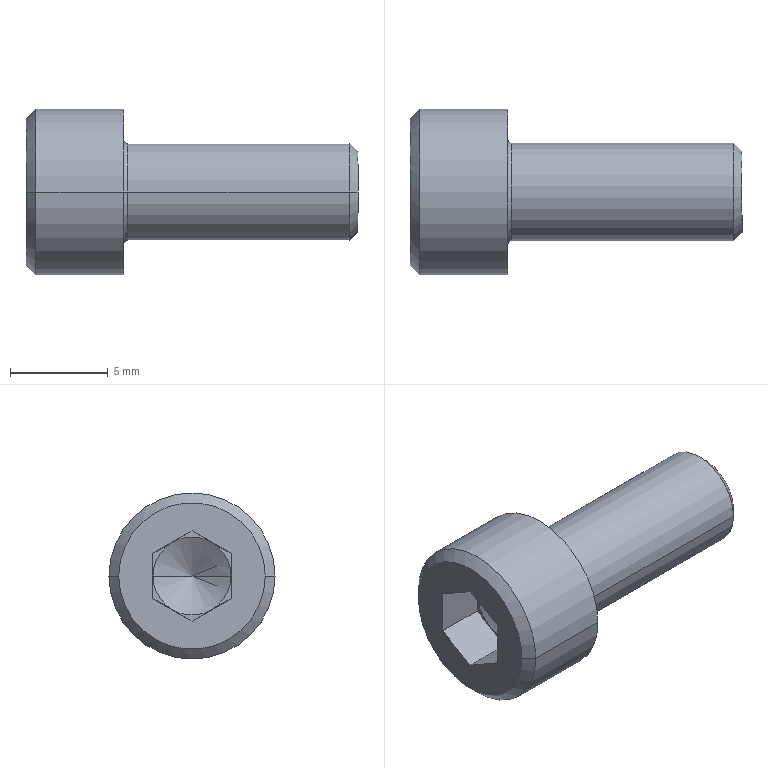Component | SolidWorks | ServoDriveMotorModule-1_MCOCGWK38_16_16-1_M5-1 | 1 solid | 27 faces | box 17 x 8.5 x 8.5 mm | volume 475 mm3 | plane 15 | cone 6 | cylinder 4 | torus 2 | commonest cylinder face diameters 8.5 x2 5 x2 | material AISI 1045 Steel, cold drawn
build123d program:
from build123d import *

# Parameters (mm, degrees)
CUT_EXTRUDE1_DEPTH = 2.5


with BuildPart() as part:
    # Sketch1 → Revolve1 (revolve)
    with BuildSketch(Plane.XY, mode=Mode.PRIVATE) as revolve1_sk:
        with BuildLine():
            Line((-5, 0), (-5, 3.75))
            Line((-5, 3.75), (-4.5, 4.25))
            Line((-4.5, 4.25), (0, 4.25))
            Line((0, 4.25), (0, 2.7))
            ThreePointArc((0, 2.7), (0.05858, 2.559), (0.2, 2.5))
            Line((0.2, 2.5), (11.567, 2.5))
            Line((11.567, 2.5), (12, 2.067))
            Line((12, 2.067), (12, 0))
            Line((12, 0), (-5, 0))
        make_face()
    revolve(revolve1_sk.sketch.rotate(Axis((12, 0, 0), (-1, 0, 0)), 270), axis=Axis((12, 0, 0), (-1, 0, 0)))

    # Sketch2 → Cut-Extrude1 (cut)
    with BuildSketch(Plane(origin=(-5, 0, 0), x_dir=(0, 0, -1), z_dir=(1, 0, 0))):
        Polygon((-2, 1.155), (-2, -1.155), (0, -2.309), (2, -1.155), (2, 1.155), (0, 2.309), align=None)
    extrude(amount=CUT_EXTRUDE1_DEPTH, mode=Mode.SUBTRACT)

    # Sketch3 → Cut-Revolve1 (revolve, cut)
    with BuildSketch(Plane.XY, mode=Mode.PRIVATE) as cut_revolve1_sk:
        Polygon((-2.5, 0), (-2.5, 2), (-1.345, 0), align=None)
    revolve(cut_revolve1_sk.sketch.rotate(Axis((-1.345, 0, 0), (-1, 0, 0)), 270), axis=Axis((-1.345, 0, 0), (-1, 0, 0)), mode=Mode.SUBTRACT)


solid = part.part

# Placed as in the assembly
solid = solid.moved(Location((-8.4, -11.5, 109), (90, 0, 0)))
STEP:
#1=COLOUR_RGB('',0.7922,0.8196,0.9333);
#2=FILL_AREA_STYLE_COLOUR('',#1);
#3=FILL_AREA_STYLE('',(#2));
#4=SURFACE_STYLE_FILL_AREA(#3);
#5=SURFACE_SIDE_STYLE('',(#4));
#6=SURFACE_STYLE_USAGE(.BOTH.,#5);
#7=PRESENTATION_STYLE_ASSIGNMENT((#6));
#8=CARTESIAN_POINT('',(-0.3837,-0.4528,4.291));
#9=VERTEX_POINT('',#8);
#10=CARTESIAN_POINT('',(-0.4291,-0.374,4.291));
#11=VERTEX_POINT('',#10);
#12=CARTESIAN_POINT('',(-0.3837,-0.4528,4.291));
#13=DIRECTION('',(-0.5,0.866,0.));
#14=VECTOR('',#13,39.37);
#15=LINE('',#12,#14);
#16=EDGE_CURVE('',#9,#11,#15,.T.);
#17=ORIENTED_EDGE('',*,*,#16,.F.);
#18=CARTESIAN_POINT('',(-0.4291,-0.5315,4.291));
#19=VERTEX_POINT('',#18);
#20=CARTESIAN_POINT('',(-0.3837,-0.4528,4.291));
#21=DIRECTION('',(-0.5,-0.866,-0.));
#22=VECTOR('',#21,39.37);
#23=LINE('',#20,#22);
#24=EDGE_CURVE('',#9,#19,#23,.T.);
#25=ORIENTED_EDGE('',*,*,#24,.T.);
#26=CARTESIAN_POINT('',(-0.4291,-0.4921,4.36));
#27=VERTEX_POINT('',#26);
#28=CARTESIAN_POINT('',(-0.4291,-0.4528,4.291));
#29=DIRECTION('',(-1.,-0.,0.));
#30=DIRECTION('',(-0.,1.,0.));
#31=AXIS2_PLACEMENT_3D('',#28,#29,#30);
#32=CIRCLE('',#31,0.07874);
#33=EDGE_CURVE('',#19,#27,#32,.T.);
#34=ORIENTED_EDGE('',*,*,#33,.T.);
#35=CARTESIAN_POINT('',(-0.4291,-0.4134,4.36));
#36=VERTEX_POINT('',#35);
#37=CARTESIAN_POINT('',(-0.4291,-0.4528,4.291));
#38=DIRECTION('',(-1.,-0.,0.));
#39=DIRECTION('',(-0.,1.,0.));
#40=AXIS2_PLACEMENT_3D('',#37,#38,#39);
#41=CIRCLE('',#40,0.07874);
#42=EDGE_CURVE('',#27,#36,#41,.T.);
#43=ORIENTED_EDGE('',*,*,#42,.T.);
#44=CARTESIAN_POINT('',(-0.4291,-0.4528,4.291));
#45=DIRECTION('',(-1.,-0.,0.));
#46=DIRECTION('',(-0.,1.,0.));
#47=AXIS2_PLACEMENT_3D('',#44,#45,#46);
#48=CIRCLE('',#47,0.07874);
#49=EDGE_CURVE('',#36,#11,#48,.T.);
#50=ORIENTED_EDGE('',*,*,#49,.T.);
#51=EDGE_LOOP('',(#17,#25,#34,#43,#50));
#52=FACE_OUTER_BOUND('',#51,.T.);
#53=CARTESIAN_POINT('',(-39.754,-0.4528,4.291));
#54=DIRECTION('',(-1.,-0.,0.));
#55=DIRECTION('',(-0.,1.,0.));
#56=AXIS2_PLACEMENT_3D('',#53,#54,#55);
#57=CONICAL_SURFACE('',#56,68.191,1.047);
#58=ADVANCED_FACE('',(#52),#57,.F.);
#59=CARTESIAN_POINT('',(-0.5276,-0.3051,4.291));
#60=VERTEX_POINT('',#59);
#61=CARTESIAN_POINT('',(-0.5276,-0.6004,4.291));
#62=VERTEX_POINT('',#61);
#63=CARTESIAN_POINT('',(-0.5276,-0.4528,4.291));
#64=DIRECTION('',(-1.,-0.,0.));
#65=DIRECTION('',(-0.,1.,0.));
#66=AXIS2_PLACEMENT_3D('',#63,#64,#65);
#67=CIRCLE('',#66,0.1476);
#68=EDGE_CURVE('',#60,#62,#67,.T.);
#69=ORIENTED_EDGE('',*,*,#68,.F.);
#70=CARTESIAN_POINT('',(-0.5079,-0.2854,4.291));
#71=VERTEX_POINT('',#70);
#72=CARTESIAN_POINT('',(-0.5079,-0.2854,4.291));
#73=DIRECTION('',(0.7071,0.7071,-0.));
#74=VECTOR('',#73,39.37);
#75=LINE('',#72,#74);
#76=EDGE_CURVE('',#60,#71,#75,.T.);
#77=ORIENTED_EDGE('',*,*,#76,.T.);
#78=CARTESIAN_POINT('',(-0.5079,-0.6201,4.291));
#79=VERTEX_POINT('',#78);
#80=CARTESIAN_POINT('',(-0.5079,-0.4528,4.291));
#81=DIRECTION('',(-1.,-0.,0.));
#82=DIRECTION('',(-0.,1.,0.));
#83=AXIS2_PLACEMENT_3D('',#80,#81,#82);
#84=CIRCLE('',#83,0.1673);
#85=EDGE_CURVE('',#71,#79,#84,.T.);
#86=ORIENTED_EDGE('',*,*,#85,.T.);
#87=CARTESIAN_POINT('',(-0.5079,-0.6201,4.291));
#88=DIRECTION('',(0.7071,-0.7071,-0.));
#89=VECTOR('',#88,39.37);
#90=LINE('',#87,#89);
#91=EDGE_CURVE('',#62,#79,#90,.T.);
#92=ORIENTED_EDGE('',*,*,#91,.F.);
#93=EDGE_LOOP('',(#69,#77,#86,#92));
#94=FACE_OUTER_BOUND('',#93,.T.);
#95=CARTESIAN_POINT('',(-0.5079,-0.4528,4.291));
#96=DIRECTION('',(1.,0.,-0.));
#97=DIRECTION('',(0.,-1.,0.));
#98=AXIS2_PLACEMENT_3D('',#95,#96,#97);
#99=CONICAL_SURFACE('',#98,0.1673,0.7854);
#100=ADVANCED_FACE('',(#94),#99,.T.);
#101=CARTESIAN_POINT('',(-0.3307,-0.2854,4.291));
#102=VERTEX_POINT('',#101);
#103=CARTESIAN_POINT('',(-0.3307,-0.6201,4.291));
#104=VERTEX_POINT('',#103);
#105=CARTESIAN_POINT('',(-0.3307,-0.4528,4.291));
#106=DIRECTION('',(-1.,-0.,0.));
#107=DIRECTION('',(-0.,1.,0.));
#108=AXIS2_PLACEMENT_3D('',#105,#106,#107);
#109=CIRCLE('',#108,0.1673);
#110=EDGE_CURVE('',#102,#104,#109,.T.);
#111=ORIENTED_EDGE('',*,*,#110,.T.);
#112=CARTESIAN_POINT('',(0.1417,-0.6201,4.291));
#113=DIRECTION('',(-1.,-0.,0.));
#114=VECTOR('',#113,39.37);
#115=LINE('',#112,#114);
#116=EDGE_CURVE('',#104,#79,#115,.T.);
#117=ORIENTED_EDGE('',*,*,#116,.T.);
#118=ORIENTED_EDGE('',*,*,#85,.F.);
#119=CARTESIAN_POINT('',(0.1417,-0.2854,4.291));
#120=DIRECTION('',(-1.,-0.,0.));
#121=VECTOR('',#120,39.37);
#122=LINE('',#119,#121);
#123=EDGE_CURVE('',#102,#71,#122,.T.);
#124=ORIENTED_EDGE('',*,*,#123,.F.);
#125=EDGE_LOOP('',(#111,#117,#118,#124));
#126=FACE_OUTER_BOUND('',#125,.T.);
#127=CARTESIAN_POINT('',(0.1417,-0.4528,4.291));
#128=DIRECTION('',(-1.,-0.,0.));
#129=DIRECTION('',(-0.,1.,0.));
#130=AXIS2_PLACEMENT_3D('',#127,#128,#129);
#131=CYLINDRICAL_SURFACE('',#130,0.1673);
#132=ADVANCED_FACE('',(#126),#131,.T.);
#133=CARTESIAN_POINT('',(-0.3307,-0.5591,4.291));
#134=VERTEX_POINT('',#133);
#135=CARTESIAN_POINT('',(-0.3307,-0.3465,4.291));
#136=VERTEX_POINT('',#135);
#137=CARTESIAN_POINT('',(-0.3307,-0.4528,4.291));
#138=DIRECTION('',(-1.,-0.,0.));
#139=DIRECTION('',(-0.,1.,0.));
#140=AXIS2_PLACEMENT_3D('',#137,#138,#139);
#141=CIRCLE('',#140,0.1063);
#142=EDGE_CURVE('',#134,#136,#141,.T.);
#143=ORIENTED_EDGE('',*,*,#142,.F.);
#144=CARTESIAN_POINT('',(-0.3228,-0.5512,4.291));
#145=VERTEX_POINT('',#144);
#146=CARTESIAN_POINT('',(-0.3228,-0.5591,4.291));
#147=DIRECTION('',(-0.,0.,-1.));
#148=DIRECTION('',(0.,1.,0.));
#149=AXIS2_PLACEMENT_3D('',#146,#147,#148);
#150=CIRCLE('',#149,0.007874);
#151=EDGE_CURVE('',#134,#145,#150,.T.);
#152=ORIENTED_EDGE('',*,*,#151,.T.);
#153=CARTESIAN_POINT('',(-0.3228,-0.3543,4.291));
#154=VERTEX_POINT('',#153);
#155=CARTESIAN_POINT('',(-0.3228,-0.4528,4.291));
#156=DIRECTION('',(-1.,-0.,0.));
#157=DIRECTION('',(-0.,1.,0.));
#158=AXIS2_PLACEMENT_3D('',#155,#156,#157);
#159=CIRCLE('',#158,0.09843);
#160=EDGE_CURVE('',#145,#154,#159,.T.);
#161=ORIENTED_EDGE('',*,*,#160,.T.);
#162=CARTESIAN_POINT('',(-0.3228,-0.3465,4.291));
#163=DIRECTION('',(0.,-0.,1.));
#164=DIRECTION('',(1.,0.,0.));
#165=AXIS2_PLACEMENT_3D('',#162,#163,#164);
#166=CIRCLE('',#165,0.007874);
#167=EDGE_CURVE('',#136,#154,#166,.T.);
#168=ORIENTED_EDGE('',*,*,#167,.F.);
#169=EDGE_LOOP('',(#143,#152,#161,#168));
#170=FACE_OUTER_BOUND('',#169,.T.);
#171=CARTESIAN_POINT('',(-0.3228,-0.4528,4.291));
#172=DIRECTION('',(-1.,-0.,0.));
#173=DIRECTION('',(-0.,1.,-0.));
#174=AXIS2_PLACEMENT_3D('',#171,#172,#173);
#175=TOROIDAL_SURFACE('',#174,0.1063,0.007874);
#176=ADVANCED_FACE('',(#170),#175,.F.);
#177=CARTESIAN_POINT('',(0.1247,-0.3543,4.291));
#178=VERTEX_POINT('',#177);
#179=CARTESIAN_POINT('',(0.1247,-0.5512,4.291));
#180=VERTEX_POINT('',#179);
#181=CARTESIAN_POINT('',(0.1247,-0.4528,4.291));
#182=DIRECTION('',(-1.,-0.,0.));
#183=DIRECTION('',(-0.,1.,0.));
#184=AXIS2_PLACEMENT_3D('',#181,#182,#183);
#185=CIRCLE('',#184,0.09843);
#186=EDGE_CURVE('',#178,#180,#185,.T.);
#187=ORIENTED_EDGE('',*,*,#186,.T.);
#188=CARTESIAN_POINT('',(0.1417,-0.5512,4.291));
#189=DIRECTION('',(-1.,-0.,0.));
#190=VECTOR('',#189,39.37);
#191=LINE('',#188,#190);
#192=EDGE_CURVE('',#180,#145,#191,.T.);
#193=ORIENTED_EDGE('',*,*,#192,.T.);
#194=CARTESIAN_POINT('',(-0.3228,-0.4528,4.291));
#195=DIRECTION('',(-1.,-0.,0.));
#196=DIRECTION('',(-0.,1.,0.));
#197=AXIS2_PLACEMENT_3D('',#194,#195,#196);
#198=CIRCLE('',#197,0.09843);
#199=EDGE_CURVE('',#154,#145,#198,.T.);
#200=ORIENTED_EDGE('',*,*,#199,.F.);
#201=CARTESIAN_POINT('',(0.1417,-0.3543,4.291));
#202=DIRECTION('',(-1.,-0.,0.));
#203=VECTOR('',#202,39.37);
#204=LINE('',#201,#203);
#205=EDGE_CURVE('',#178,#154,#204,.T.);
#206=ORIENTED_EDGE('',*,*,#205,.F.);
#207=EDGE_LOOP('',(#187,#193,#200,#206));
#208=FACE_OUTER_BOUND('',#207,.T.);
#209=CARTESIAN_POINT('',(0.1417,-0.4528,4.291));
#210=DIRECTION('',(-1.,-0.,0.));
#211=DIRECTION('',(-0.,1.,0.));
#212=AXIS2_PLACEMENT_3D('',#209,#210,#211);
#213=CYLINDRICAL_SURFACE('',#212,0.09843);
#214=ADVANCED_FACE('',(#208),#213,.T.);
#215=CARTESIAN_POINT('',(0.1417,-0.3714,4.291));
#216=VERTEX_POINT('',#215);
#217=CARTESIAN_POINT('',(0.1417,-0.5341,4.291));
#218=VERTEX_POINT('',#217);
#219=CARTESIAN_POINT('',(0.1417,-0.4528,4.291));
#220=DIRECTION('',(-1.,-0.,0.));
#221=DIRECTION('',(-0.,1.,0.));
#222=AXIS2_PLACEMENT_3D('',#219,#220,#221);
#223=CIRCLE('',#222,0.08138);
#224=EDGE_CURVE('',#216,#218,#223,.T.);
#225=ORIENTED_EDGE('',*,*,#224,.T.);
#226=CARTESIAN_POINT('',(0.1417,-0.5341,4.291));
#227=DIRECTION('',(-0.7071,-0.7071,-0.));
#228=VECTOR('',#227,39.37);
#229=LINE('',#226,#228);
#230=EDGE_CURVE('',#218,#180,#229,.T.);
#231=ORIENTED_EDGE('',*,*,#230,.T.);
#232=ORIENTED_EDGE('',*,*,#186,.F.);
#233=CARTESIAN_POINT('',(0.1417,-0.3714,4.291));
#234=DIRECTION('',(-0.7071,0.7071,0.));
#235=VECTOR('',#234,39.37);
#236=LINE('',#233,#235);
#237=EDGE_CURVE('',#216,#178,#236,.T.);
#238=ORIENTED_EDGE('',*,*,#237,.F.);
#239=EDGE_LOOP('',(#225,#231,#232,#238));
#240=FACE_OUTER_BOUND('',#239,.T.);
#241=CARTESIAN_POINT('',(0.1417,-0.4528,4.291));
#242=DIRECTION('',(-1.,-0.,0.));
#243=DIRECTION('',(-0.,1.,0.));
#244=AXIS2_PLACEMENT_3D('',#241,#242,#243);
#245=CONICAL_SURFACE('',#244,0.08138,0.7854);
#246=ADVANCED_FACE('',(#240),#245,.T.);
#247=CARTESIAN_POINT('',(-0.4291,-0.4134,4.223));
#248=VERTEX_POINT('',#247);
#249=CARTESIAN_POINT('',(-0.4291,-0.4528,4.291));
#250=DIRECTION('',(-1.,-0.,0.));
#251=DIRECTION('',(-0.,1.,0.));
#252=AXIS2_PLACEMENT_3D('',#249,#250,#251);
#253=CIRCLE('',#252,0.07874);
#254=EDGE_CURVE('',#11,#248,#253,.T.);
#255=ORIENTED_EDGE('',*,*,#254,.F.);
#256=CARTESIAN_POINT('',(-0.4291,-0.374,4.246));
#257=VERTEX_POINT('',#256);
#258=CARTESIAN_POINT('',(-0.4291,-0.374,4.246));
#259=DIRECTION('',(0.,-0.,1.));
#260=VECTOR('',#259,39.37);
#261=LINE('',#258,#260);
#262=EDGE_CURVE('',#257,#11,#261,.T.);
#263=ORIENTED_EDGE('',*,*,#262,.F.);
#264=CARTESIAN_POINT('',(-0.4291,-0.4528,4.2));
#265=DIRECTION('',(-0.,0.866,0.5));
#266=VECTOR('',#265,39.37);
#267=LINE('',#264,#266);
#268=EDGE_CURVE('',#248,#257,#267,.T.);
#269=ORIENTED_EDGE('',*,*,#268,.F.);
#270=EDGE_LOOP('',(#255,#263,#269));
#271=FACE_OUTER_BOUND('',#270,.T.);
#272=CARTESIAN_POINT('',(-0.4291,-0.4528,4.291));
#273=DIRECTION('',(1.,0.,-0.));
#274=DIRECTION('',(0.,-1.,-0.));
#275=AXIS2_PLACEMENT_3D('',#272,#273,#274);
#276=PLANE('',#275);
#277=ADVANCED_FACE('',(#271),#276,.F.);
#278=CARTESIAN_POINT('',(-0.4291,-0.4921,4.223));
#279=VERTEX_POINT('',#278);
#280=CARTESIAN_POINT('',(-0.4291,-0.4528,4.291));
#281=DIRECTION('',(-1.,-0.,0.));
#282=DIRECTION('',(-0.,1.,0.));
#283=AXIS2_PLACEMENT_3D('',#280,#281,#282);
#284=CIRCLE('',#283,0.07874);
#285=EDGE_CURVE('',#248,#279,#284,.T.);
#286=ORIENTED_EDGE('',*,*,#285,.F.);
#287=CARTESIAN_POINT('',(-0.4291,-0.4528,4.2));
#288=VERTEX_POINT('',#287);
#289=CARTESIAN_POINT('',(-0.4291,-0.4528,4.2));
#290=DIRECTION('',(-0.,0.866,0.5));
#291=VECTOR('',#290,39.37);
#292=LINE('',#289,#291);
#293=EDGE_CURVE('',#288,#248,#292,.T.);
#294=ORIENTED_EDGE('',*,*,#293,.F.);
#295=CARTESIAN_POINT('',(-0.4291,-0.5315,4.246));
#296=DIRECTION('',(-0.,0.866,-0.5));
#297=VECTOR('',#296,39.37);
#298=LINE('',#295,#297);
#299=EDGE_CURVE('',#279,#288,#298,.T.);
#300=ORIENTED_EDGE('',*,*,#299,.F.);
#301=EDGE_LOOP('',(#286,#294,#300));
#302=FACE_OUTER_BOUND('',#301,.T.);
#303=CARTESIAN_POINT('',(-0.4291,-0.4528,4.291));
#304=DIRECTION('',(1.,0.,-0.));
#305=DIRECTION('',(0.,-1.,-0.));
#306=AXIS2_PLACEMENT_3D('',#303,#304,#305);
#307=PLANE('',#306);
#308=ADVANCED_FACE('',(#302),#307,.F.);
#309=CARTESIAN_POINT('',(-0.4291,-0.4528,4.291));
#310=DIRECTION('',(-1.,-0.,0.));
#311=DIRECTION('',(-0.,1.,0.));
#312=AXIS2_PLACEMENT_3D('',#309,#310,#311);
#313=CIRCLE('',#312,0.07874);
#314=EDGE_CURVE('',#279,#19,#313,.T.);
#315=ORIENTED_EDGE('',*,*,#314,.F.);
#316=CARTESIAN_POINT('',(-0.4291,-0.5315,4.246));
#317=VERTEX_POINT('',#316);
#318=CARTESIAN_POINT('',(-0.4291,-0.5315,4.246));
#319=DIRECTION('',(-0.,0.866,-0.5));
#320=VECTOR('',#319,39.37);
#321=LINE('',#318,#320);
#322=EDGE_CURVE('',#317,#279,#321,.T.);
#323=ORIENTED_EDGE('',*,*,#322,.F.);
#324=CARTESIAN_POINT('',(-0.4291,-0.5315,4.337));
#325=DIRECTION('',(-0.,0.,-1.));
#326=VECTOR('',#325,39.37);
#327=LINE('',#324,#326);
#328=EDGE_CURVE('',#19,#317,#327,.T.);
#329=ORIENTED_EDGE('',*,*,#328,.F.);
#330=EDGE_LOOP('',(#315,#323,#329));
#331=FACE_OUTER_BOUND('',#330,.T.);
#332=CARTESIAN_POINT('',(-0.4291,-0.4528,4.291));
#333=DIRECTION('',(1.,0.,-0.));
#334=DIRECTION('',(0.,-1.,-0.));
#335=AXIS2_PLACEMENT_3D('',#332,#333,#334);
#336=PLANE('',#335);
#337=ADVANCED_FACE('',(#331),#336,.F.);
#338=ORIENTED_EDGE('',*,*,#33,.F.);
#339=CARTESIAN_POINT('',(-0.4291,-0.5315,4.337));
#340=VERTEX_POINT('',#339);
#341=CARTESIAN_POINT('',(-0.4291,-0.5315,4.337));
#342=DIRECTION('',(-0.,0.,-1.));
#343=VECTOR('',#342,39.37);
#344=LINE('',#341,#343);
#345=EDGE_CURVE('',#340,#19,#344,.T.);
#346=ORIENTED_EDGE('',*,*,#345,.F.);
#347=CARTESIAN_POINT('',(-0.4291,-0.4528,4.382));
#348=DIRECTION('',(0.,-0.866,-0.5));
#349=VECTOR('',#348,39.37);
#350=LINE('',#347,#349);
#351=EDGE_CURVE('',#27,#340,#350,.T.);
#352=ORIENTED_EDGE('',*,*,#351,.F.);
#353=EDGE_LOOP('',(#338,#346,#352));
#354=FACE_OUTER_BOUND('',#353,.T.);
#355=CARTESIAN_POINT('',(-0.4291,-0.4528,4.291));
#356=DIRECTION('',(1.,0.,-0.));
#357=DIRECTION('',(0.,-1.,-0.));
#358=AXIS2_PLACEMENT_3D('',#355,#356,#357);
#359=PLANE('',#358);
#360=ADVANCED_FACE('',(#354),#359,.F.);
#361=ORIENTED_EDGE('',*,*,#42,.F.);
#362=CARTESIAN_POINT('',(-0.4291,-0.4528,4.382));
#363=VERTEX_POINT('',#362);
#364=CARTESIAN_POINT('',(-0.4291,-0.4528,4.382));
#365=DIRECTION('',(0.,-0.866,-0.5));
#366=VECTOR('',#365,39.37);
#367=LINE('',#364,#366);
#368=EDGE_CURVE('',#363,#27,#367,.T.);
#369=ORIENTED_EDGE('',*,*,#368,.F.);
#370=CARTESIAN_POINT('',(-0.4291,-0.374,4.337));
#371=DIRECTION('',(0.,-0.866,0.5));
#372=VECTOR('',#371,39.37);
#373=LINE('',#370,#372);
#374=EDGE_CURVE('',#36,#363,#373,.T.);
#375=ORIENTED_EDGE('',*,*,#374,.F.);
#376=EDGE_LOOP('',(#361,#369,#375));
#377=FACE_OUTER_BOUND('',#376,.T.);
#378=CARTESIAN_POINT('',(-0.4291,-0.4528,4.291));
#379=DIRECTION('',(1.,0.,-0.));
#380=DIRECTION('',(0.,-1.,-0.));
#381=AXIS2_PLACEMENT_3D('',#378,#379,#380);
#382=PLANE('',#381);
#383=ADVANCED_FACE('',(#377),#382,.F.);
#384=ORIENTED_EDGE('',*,*,#49,.F.);
#385=CARTESIAN_POINT('',(-0.4291,-0.374,4.337));
#386=VERTEX_POINT('',#385);
#387=CARTESIAN_POINT('',(-0.4291,-0.374,4.337));
#388=DIRECTION('',(0.,-0.866,0.5));
#389=VECTOR('',#388,39.37);
#390=LINE('',#387,#389);
#391=EDGE_CURVE('',#386,#36,#390,.T.);
#392=ORIENTED_EDGE('',*,*,#391,.F.);
#393=CARTESIAN_POINT('',(-0.4291,-0.374,4.246));
#394=DIRECTION('',(0.,-0.,1.));
#395=VECTOR('',#394,39.37);
#396=LINE('',#393,#395);
#397=EDGE_CURVE('',#11,#386,#396,.T.);
#398=ORIENTED_EDGE('',*,*,#397,.F.);
#399=EDGE_LOOP('',(#384,#392,#398));
#400=FACE_OUTER_BOUND('',#399,.T.);
#401=CARTESIAN_POINT('',(-0.4291,-0.4528,4.291));
#402=DIRECTION('',(1.,0.,-0.));
#403=DIRECTION('',(0.,-1.,-0.));
#404=AXIS2_PLACEMENT_3D('',#401,#402,#403);
#405=PLANE('',#404);
#406=ADVANCED_FACE('',(#400),#405,.F.);
#407=CARTESIAN_POINT('',(-0.5276,-0.4528,4.291));
#408=DIRECTION('',(-1.,-0.,0.));
#409=DIRECTION('',(-0.,1.,0.));
#410=AXIS2_PLACEMENT_3D('',#407,#408,#409);
#411=CIRCLE('',#410,0.1476);
#412=EDGE_CURVE('',#62,#60,#411,.T.);
#413=ORIENTED_EDGE('',*,*,#412,.T.);
#414=ORIENTED_EDGE('',*,*,#68,.T.);
#415=EDGE_LOOP('',(#413,#414));
#416=FACE_OUTER_BOUND('',#415,.T.);
#417=CARTESIAN_POINT('',(-0.5276,-0.4528,4.2));
#418=VERTEX_POINT('',#417);
#419=CARTESIAN_POINT('',(-0.5276,-0.374,4.246));
#420=VERTEX_POINT('',#419);
#421=CARTESIAN_POINT('',(-0.5276,-0.4528,4.2));
#422=DIRECTION('',(-0.,0.866,0.5));
#423=VECTOR('',#422,39.37);
#424=LINE('',#421,#423);
#425=EDGE_CURVE('',#418,#420,#424,.T.);
#426=ORIENTED_EDGE('',*,*,#425,.T.);
#427=CARTESIAN_POINT('',(-0.5276,-0.374,4.337));
#428=VERTEX_POINT('',#427);
#429=CARTESIAN_POINT('',(-0.5276,-0.374,4.246));
#430=DIRECTION('',(0.,-0.,1.));
#431=VECTOR('',#430,39.37);
#432=LINE('',#429,#431);
#433=EDGE_CURVE('',#420,#428,#432,.T.);
#434=ORIENTED_EDGE('',*,*,#433,.T.);
#435=CARTESIAN_POINT('',(-0.5276,-0.4528,4.382));
#436=VERTEX_POINT('',#435);
#437=CARTESIAN_POINT('',(-0.5276,-0.374,4.337));
#438=DIRECTION('',(0.,-0.866,0.5));
#439=VECTOR('',#438,39.37);
#440=LINE('',#437,#439);
#441=EDGE_CURVE('',#428,#436,#440,.T.);
#442=ORIENTED_EDGE('',*,*,#441,.T.);
#443=CARTESIAN_POINT('',(-0.5276,-0.5315,4.337));
#444=VERTEX_POINT('',#443);
#445=CARTESIAN_POINT('',(-0.5276,-0.4528,4.382));
#446=DIRECTION('',(0.,-0.866,-0.5));
#447=VECTOR('',#446,39.37);
#448=LINE('',#445,#447);
#449=EDGE_CURVE('',#436,#444,#448,.T.);
#450=ORIENTED_EDGE('',*,*,#449,.T.);
#451=CARTESIAN_POINT('',(-0.5276,-0.5315,4.246));
#452=VERTEX_POINT('',#451);
#453=CARTESIAN_POINT('',(-0.5276,-0.5315,4.337));
#454=DIRECTION('',(-0.,0.,-1.));
#455=VECTOR('',#454,39.37);
#456=LINE('',#453,#455);
#457=EDGE_CURVE('',#444,#452,#456,.T.);
#458=ORIENTED_EDGE('',*,*,#457,.T.);
#459=CARTESIAN_POINT('',(-0.5276,-0.5315,4.246));
#460=DIRECTION('',(-0.,0.866,-0.5));
#461=VECTOR('',#460,39.37);
#462=LINE('',#459,#461);
#463=EDGE_CURVE('',#452,#418,#462,.T.);
#464=ORIENTED_EDGE('',*,*,#463,.T.);
#465=EDGE_LOOP('',(#426,#434,#442,#450,#458,#464));
#466=FACE_BOUND('',#465,.T.);
#467=CARTESIAN_POINT('',(-0.5276,-0.4528,4.291));
#468=DIRECTION('',(1.,0.,-0.));
#469=DIRECTION('',(0.,-1.,-0.));
#470=AXIS2_PLACEMENT_3D('',#467,#468,#469);
#471=PLANE('',#470);
#472=ADVANCED_FACE('',(#416,#466),#471,.F.);
#473=ORIENTED_EDGE('',*,*,#224,.F.);
#474=CARTESIAN_POINT('',(0.1417,-0.4528,4.291));
#475=DIRECTION('',(-1.,-0.,0.));
#476=DIRECTION('',(-0.,1.,0.));
#477=AXIS2_PLACEMENT_3D('',#474,#475,#476);
#478=CIRCLE('',#477,0.08138);
#479=EDGE_CURVE('',#218,#216,#478,.T.);
#480=ORIENTED_EDGE('',*,*,#479,.F.);
#481=EDGE_LOOP('',(#473,#480));
#482=FACE_OUTER_BOUND('',#481,.T.);
#483=CARTESIAN_POINT('',(0.1417,-0.4528,4.21));
#484=DIRECTION('',(-1.,-0.,0.));
#485=DIRECTION('',(-0.,1.,0.));
#486=AXIS2_PLACEMENT_3D('',#483,#484,#485);
#487=PLANE('',#486);
#488=ADVANCED_FACE('',(#482),#487,.F.);
#489=ORIENTED_EDGE('',*,*,#230,.F.);
#490=ORIENTED_EDGE('',*,*,#479,.T.);
#491=ORIENTED_EDGE('',*,*,#237,.T.);
#492=CARTESIAN_POINT('',(0.1247,-0.4528,4.291));
#493=DIRECTION('',(-1.,-0.,0.));
#494=DIRECTION('',(-0.,1.,0.));
#495=AXIS2_PLACEMENT_3D('',#492,#493,#494);
#496=CIRCLE('',#495,0.09843);
#497=EDGE_CURVE('',#180,#178,#496,.T.);
#498=ORIENTED_EDGE('',*,*,#497,.F.);
#499=EDGE_LOOP('',(#489,#490,#491,#498));
#500=FACE_OUTER_BOUND('',#499,.T.);
#501=CARTESIAN_POINT('',(0.1417,-0.4528,4.291));
#502=DIRECTION('',(-1.,-0.,0.));
#503=DIRECTION('',(-0.,1.,0.));
#504=AXIS2_PLACEMENT_3D('',#501,#502,#503);
#505=CONICAL_SURFACE('',#504,0.08138,0.7854);
#506=ADVANCED_FACE('',(#500),#505,.T.);
#507=ORIENTED_EDGE('',*,*,#192,.F.);
#508=ORIENTED_EDGE('',*,*,#497,.T.);
#509=ORIENTED_EDGE('',*,*,#205,.T.);
#510=ORIENTED_EDGE('',*,*,#160,.F.);
#511=EDGE_LOOP('',(#507,#508,#509,#510));
#512=FACE_OUTER_BOUND('',#511,.T.);
#513=CARTESIAN_POINT('',(0.1417,-0.4528,4.291));
#514=DIRECTION('',(-1.,-0.,0.));
#515=DIRECTION('',(-0.,1.,0.));
#516=AXIS2_PLACEMENT_3D('',#513,#514,#515);
#517=CYLINDRICAL_SURFACE('',#516,0.09843);
#518=ADVANCED_FACE('',(#512),#517,.T.);
#519=ORIENTED_EDGE('',*,*,#151,.F.);
#520=CARTESIAN_POINT('',(-0.3307,-0.4528,4.291));
#521=DIRECTION('',(-1.,-0.,0.));
#522=DIRECTION('',(-0.,1.,0.));
#523=AXIS2_PLACEMENT_3D('',#520,#521,#522);
#524=CIRCLE('',#523,0.1063);
#525=EDGE_CURVE('',#136,#134,#524,.T.);
#526=ORIENTED_EDGE('',*,*,#525,.F.);
#527=ORIENTED_EDGE('',*,*,#167,.T.);
#528=ORIENTED_EDGE('',*,*,#199,.T.);
#529=EDGE_LOOP('',(#519,#526,#527,#528));
#530=FACE_OUTER_BOUND('',#529,.T.);
#531=CARTESIAN_POINT('',(-0.3228,-0.4528,4.291));
#532=DIRECTION('',(-1.,-0.,0.));
#533=DIRECTION('',(-0.,1.,-0.));
#534=AXIS2_PLACEMENT_3D('',#531,#532,#533);
#535=TOROIDAL_SURFACE('',#534,0.1063,0.007874);
#536=ADVANCED_FACE('',(#530),#535,.F.);
#537=ORIENTED_EDGE('',*,*,#110,.F.);
#538=CARTESIAN_POINT('',(-0.3307,-0.4528,4.291));
#539=DIRECTION('',(-1.,-0.,0.));
#540=DIRECTION('',(-0.,1.,0.));
#541=AXIS2_PLACEMENT_3D('',#538,#539,#540);
#542=CIRCLE('',#541,0.1673);
#543=EDGE_CURVE('',#104,#102,#542,.T.);
#544=ORIENTED_EDGE('',*,*,#543,.F.);
#545=EDGE_LOOP('',(#537,#544));
#546=FACE_OUTER_BOUND('',#545,.T.);
#547=ORIENTED_EDGE('',*,*,#525,.T.);
#548=ORIENTED_EDGE('',*,*,#142,.T.);
#549=EDGE_LOOP('',(#547,#548));
#550=FACE_BOUND('',#549,.T.);
#551=CARTESIAN_POINT('',(-0.3307,-0.4528,4.124));
#552=DIRECTION('',(-1.,-0.,0.));
#553=DIRECTION('',(-0.,1.,0.));
#554=AXIS2_PLACEMENT_3D('',#551,#552,#553);
#555=PLANE('',#554);
#556=ADVANCED_FACE('',(#546,#550),#555,.F.);
#557=ORIENTED_EDGE('',*,*,#116,.F.);
#558=ORIENTED_EDGE('',*,*,#543,.T.);
#559=ORIENTED_EDGE('',*,*,#123,.T.);
#560=CARTESIAN_POINT('',(-0.5079,-0.4528,4.291));
#561=DIRECTION('',(-1.,-0.,0.));
#562=DIRECTION('',(-0.,1.,0.));
#563=AXIS2_PLACEMENT_3D('',#560,#561,#562);
#564=CIRCLE('',#563,0.1673);
#565=EDGE_CURVE('',#79,#71,#564,.T.);
#566=ORIENTED_EDGE('',*,*,#565,.F.);
#567=EDGE_LOOP('',(#557,#558,#559,#566));
#568=FACE_OUTER_BOUND('',#567,.T.);
#569=CARTESIAN_POINT('',(0.1417,-0.4528,4.291));
#570=DIRECTION('',(-1.,-0.,0.));
#571=DIRECTION('',(-0.,1.,0.));
#572=AXIS2_PLACEMENT_3D('',#569,#570,#571);
#573=CYLINDRICAL_SURFACE('',#572,0.1673);
#574=ADVANCED_FACE('',(#568),#573,.T.);
#575=ORIENTED_EDGE('',*,*,#76,.F.);
#576=ORIENTED_EDGE('',*,*,#412,.F.);
#577=ORIENTED_EDGE('',*,*,#91,.T.);
#578=ORIENTED_EDGE('',*,*,#565,.T.);
#579=EDGE_LOOP('',(#575,#576,#577,#578));
#580=FACE_OUTER_BOUND('',#579,.T.);
#581=CARTESIAN_POINT('',(-0.5079,-0.4528,4.291));
#582=DIRECTION('',(1.,0.,-0.));
#583=DIRECTION('',(0.,-1.,0.));
#584=AXIS2_PLACEMENT_3D('',#581,#582,#583);
#585=CONICAL_SURFACE('',#584,0.1673,0.7854);
#586=ADVANCED_FACE('',(#580),#585,.T.);
#587=ORIENTED_EDGE('',*,*,#425,.F.);
#588=CARTESIAN_POINT('',(-0.4291,-0.4528,4.2));
#589=DIRECTION('',(-1.,-0.,0.));
#590=VECTOR('',#589,39.37);
#591=LINE('',#588,#590);
#592=EDGE_CURVE('',#288,#418,#591,.T.);
#593=ORIENTED_EDGE('',*,*,#592,.F.);
#594=ORIENTED_EDGE('',*,*,#293,.T.);
#595=ORIENTED_EDGE('',*,*,#268,.T.);
#596=CARTESIAN_POINT('',(-0.4291,-0.374,4.246));
#597=DIRECTION('',(-1.,-0.,0.));
#598=VECTOR('',#597,39.37);
#599=LINE('',#596,#598);
#600=EDGE_CURVE('',#257,#420,#599,.T.);
#601=ORIENTED_EDGE('',*,*,#600,.T.);
#602=EDGE_LOOP('',(#587,#593,#594,#595,#601));
#603=FACE_OUTER_BOUND('',#602,.T.);
#604=CARTESIAN_POINT('',(-0.4291,-0.4528,4.2));
#605=DIRECTION('',(0.,-0.5,0.866));
#606=DIRECTION('',(0.,-0.866,-0.5));
#607=AXIS2_PLACEMENT_3D('',#604,#605,#606);
#608=PLANE('',#607);
#609=ADVANCED_FACE('',(#603),#608,.T.);
#610=ORIENTED_EDGE('',*,*,#433,.F.);
#611=ORIENTED_EDGE('',*,*,#600,.F.);
#612=ORIENTED_EDGE('',*,*,#262,.T.);
#613=ORIENTED_EDGE('',*,*,#397,.T.);
#614=CARTESIAN_POINT('',(-0.4291,-0.374,4.337));
#615=DIRECTION('',(-1.,-0.,0.));
#616=VECTOR('',#615,39.37);
#617=LINE('',#614,#616);
#618=EDGE_CURVE('',#386,#428,#617,.T.);
#619=ORIENTED_EDGE('',*,*,#618,.T.);
#620=EDGE_LOOP('',(#610,#611,#612,#613,#619));
#621=FACE_OUTER_BOUND('',#620,.T.);
#622=CARTESIAN_POINT('',(-0.4291,-0.374,4.246));
#623=DIRECTION('',(0.,-1.,-0.));
#624=DIRECTION('',(-1.,-0.,0.));
#625=AXIS2_PLACEMENT_3D('',#622,#623,#624);
#626=PLANE('',#625);
#627=ADVANCED_FACE('',(#621),#626,.T.);
#628=ORIENTED_EDGE('',*,*,#441,.F.);
#629=ORIENTED_EDGE('',*,*,#618,.F.);
#630=ORIENTED_EDGE('',*,*,#391,.T.);
#631=ORIENTED_EDGE('',*,*,#374,.T.);
#632=CARTESIAN_POINT('',(-0.4291,-0.4528,4.382));
#633=DIRECTION('',(-1.,-0.,0.));
#634=VECTOR('',#633,39.37);
#635=LINE('',#632,#634);
#636=EDGE_CURVE('',#363,#436,#635,.T.);
#637=ORIENTED_EDGE('',*,*,#636,.T.);
#638=EDGE_LOOP('',(#628,#629,#630,#631,#637));
#639=FACE_OUTER_BOUND('',#638,.T.);
#640=CARTESIAN_POINT('',(-0.4291,-0.374,4.337));
#641=DIRECTION('',(0.,-0.5,-0.866));
#642=DIRECTION('',(-0.,0.866,-0.5));
#643=AXIS2_PLACEMENT_3D('',#640,#641,#642);
#644=PLANE('',#643);
#645=ADVANCED_FACE('',(#639),#644,.T.);
#646=ORIENTED_EDGE('',*,*,#449,.F.);
#647=ORIENTED_EDGE('',*,*,#636,.F.);
#648=ORIENTED_EDGE('',*,*,#368,.T.);
#649=ORIENTED_EDGE('',*,*,#351,.T.);
#650=CARTESIAN_POINT('',(-0.4291,-0.5315,4.337));
#651=DIRECTION('',(-1.,-0.,0.));
#652=VECTOR('',#651,39.37);
#653=LINE('',#650,#652);
#654=EDGE_CURVE('',#340,#444,#653,.T.);
#655=ORIENTED_EDGE('',*,*,#654,.T.);
#656=EDGE_LOOP('',(#646,#647,#648,#649,#655));
#657=FACE_OUTER_BOUND('',#656,.T.);
#658=CARTESIAN_POINT('',(-0.4291,-0.4528,4.382));
#659=DIRECTION('',(-0.,0.5,-0.866));
#660=DIRECTION('',(-0.,0.866,0.5));
#661=AXIS2_PLACEMENT_3D('',#658,#659,#660);
#662=PLANE('',#661);
#663=ADVANCED_FACE('',(#657),#662,.T.);
#664=ORIENTED_EDGE('',*,*,#457,.F.);
#665=ORIENTED_EDGE('',*,*,#654,.F.);
#666=ORIENTED_EDGE('',*,*,#345,.T.);
#667=ORIENTED_EDGE('',*,*,#328,.T.);
#668=CARTESIAN_POINT('',(-0.4291,-0.5315,4.246));
#669=DIRECTION('',(-1.,-0.,0.));
#670=VECTOR('',#669,39.37);
#671=LINE('',#668,#670);
#672=EDGE_CURVE('',#317,#452,#671,.T.);
#673=ORIENTED_EDGE('',*,*,#672,.T.);
#674=EDGE_LOOP('',(#664,#665,#666,#667,#673));
#675=FACE_OUTER_BOUND('',#674,.T.);
#676=CARTESIAN_POINT('',(-0.4291,-0.5315,4.337));
#677=DIRECTION('',(-0.,1.,0.));
#678=DIRECTION('',(1.,0.,-0.));
#679=AXIS2_PLACEMENT_3D('',#676,#677,#678);
#680=PLANE('',#679);
#681=ADVANCED_FACE('',(#675),#680,.T.);
#682=ORIENTED_EDGE('',*,*,#463,.F.);
#683=ORIENTED_EDGE('',*,*,#672,.F.);
#684=ORIENTED_EDGE('',*,*,#322,.T.);
#685=ORIENTED_EDGE('',*,*,#299,.T.);
#686=ORIENTED_EDGE('',*,*,#592,.T.);
#687=EDGE_LOOP('',(#682,#683,#684,#685,#686));
#688=FACE_OUTER_BOUND('',#687,.T.);
#689=CARTESIAN_POINT('',(-0.4291,-0.5315,4.246));
#690=DIRECTION('',(-0.,0.5,0.866));
#691=DIRECTION('',(0.,-0.866,0.5));
#692=AXIS2_PLACEMENT_3D('',#689,#690,#691);
#693=PLANE('',#692);
#694=ADVANCED_FACE('',(#688),#693,.T.);
#695=ORIENTED_EDGE('',*,*,#24,.F.);
#696=ORIENTED_EDGE('',*,*,#16,.T.);
#697=ORIENTED_EDGE('',*,*,#254,.T.);
#698=ORIENTED_EDGE('',*,*,#285,.T.);
#699=ORIENTED_EDGE('',*,*,#314,.T.);
#700=EDGE_LOOP('',(#695,#696,#697,#698,#699));
#701=FACE_OUTER_BOUND('',#700,.T.);
#702=CARTESIAN_POINT('',(-39.754,-0.4528,4.291));
#703=DIRECTION('',(-1.,-0.,0.));
#704=DIRECTION('',(-0.,1.,0.));
#705=AXIS2_PLACEMENT_3D('',#702,#703,#704);
#706=CONICAL_SURFACE('',#705,68.191,1.047);
#707=ADVANCED_FACE('',(#701),#706,.F.);
#708=CLOSED_SHELL('',(#58,#100,#132,#176,#214,#246,#277,#308,#337,#360,#383,#406,#472,#488,#506,#518,#536,#556,#574,#586,#609,#627,#645,#663,#681,#694,#707));
#709=MANIFOLD_SOLID_BREP('',#708);
#710=STYLED_ITEM('',(#7),#709);
#711=PRESENTATION_LAYER_ASSIGNMENT('','',(#710));
#712=(LENGTH_UNIT()NAMED_UNIT(*)SI_UNIT($,.METRE.));
#713=LENGTH_MEASURE_WITH_UNIT(LENGTH_MEASURE(0.0254),#712);
#714=DIMENSIONAL_EXPONENTS(1.,0.,0.,0.,0.,0.,0.);
#715=(CONVERSION_BASED_UNIT('',#713)LENGTH_UNIT()NAMED_UNIT(#714));
#716=UNCERTAINTY_MEASURE_WITH_UNIT(LENGTH_MEASURE(0.00001),#715,'','');
#717=(NAMED_UNIT(*)PLANE_ANGLE_UNIT()SI_UNIT($,.RADIAN.));
#718=(NAMED_UNIT(*)SI_UNIT($,.STERADIAN.)SOLID_ANGLE_UNIT());
#719=(GEOMETRIC_REPRESENTATION_CONTEXT(3)GLOBAL_UNCERTAINTY_ASSIGNED_CONTEXT((#716))GLOBAL_UNIT_ASSIGNED_CONTEXT((#715,#717,#718))REPRESENTATION_CONTEXT('',''));
#720=MECHANICAL_DESIGN_GEOMETRIC_PRESENTATION_REPRESENTATION('',(#710),#719);
#721=CARTESIAN_POINT('',(0.,0.,0.));
#722=DIRECTION('',(0.,0.,1.));
#723=DIRECTION('',(1.,0.,0.));
#724=AXIS2_PLACEMENT_3D('',#721,#722,#723);
#725=(LENGTH_UNIT()NAMED_UNIT(*)SI_UNIT($,.METRE.));
#726=LENGTH_MEASURE_WITH_UNIT(LENGTH_MEASURE(0.0254),#725);
#727=DIMENSIONAL_EXPONENTS(1.,0.,0.,0.,0.,0.,0.);
#728=(CONVERSION_BASED_UNIT('',#726)LENGTH_UNIT()NAMED_UNIT(#727));
#729=UNCERTAINTY_MEASURE_WITH_UNIT(LENGTH_MEASURE(0.00001),#728,'','');
#730=(NAMED_UNIT(*)PLANE_ANGLE_UNIT()SI_UNIT($,.RADIAN.));
#731=(NAMED_UNIT(*)SI_UNIT($,.STERADIAN.)SOLID_ANGLE_UNIT());
#732=(GEOMETRIC_REPRESENTATION_CONTEXT(3)GLOBAL_UNCERTAINTY_ASSIGNED_CONTEXT((#729))GLOBAL_UNIT_ASSIGNED_CONTEXT((#728,#730,#731))REPRESENTATION_CONTEXT('',''));
#733=ADVANCED_BREP_SHAPE_REPRESENTATION('',(#709,#724),#732);